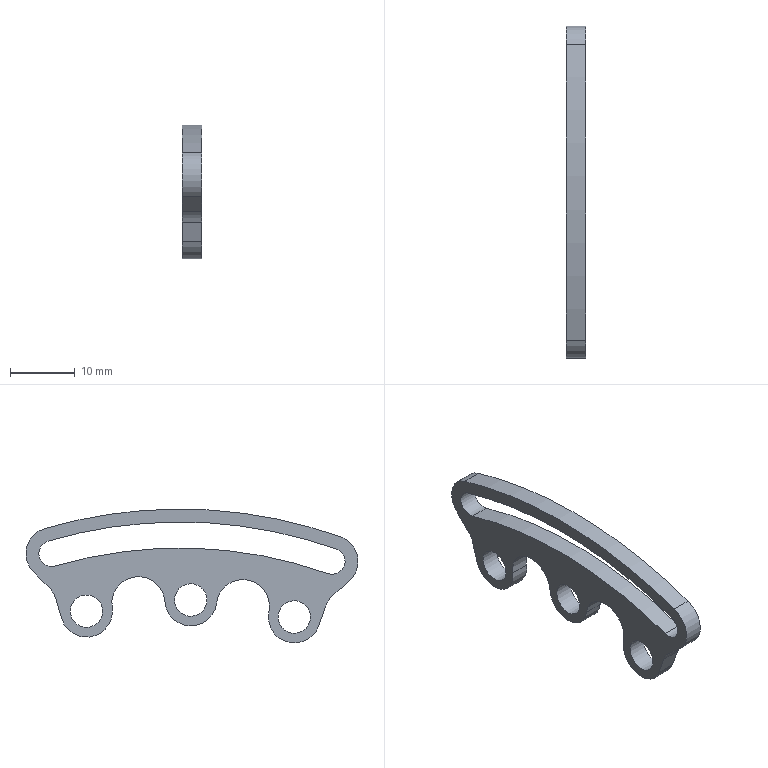Component | NX | 21__27_2 | 1 solid | 23 faces | volume 1308 mm3 | cylinder 17 | plane 6 | commonest cylinder face diameters 8 x7 5 x3 4 x2 8.2 x2 144 x1 148 x1 136 x1